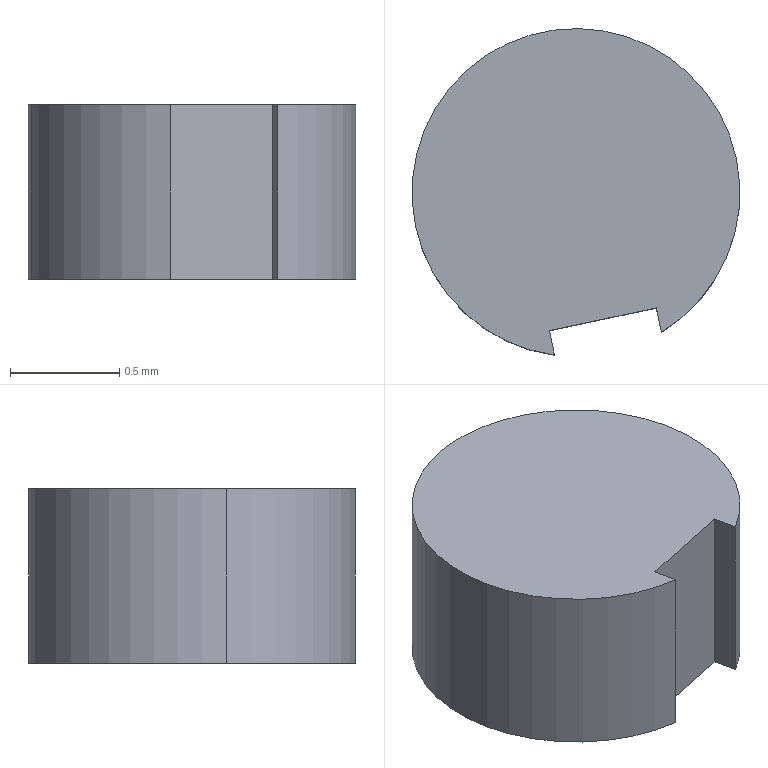Component | SolidWorks | Part32^Assembly1-2 | 1 solid | 8 faces | box 1.5 x 1.49 x 0.8 mm | volume 1 mm3 | plane 5 | cylinder 3 | commonest cylinder face diameters 1.5 x3
STEP:
#1=COLOUR_RGB('',0.7922,0.8196,0.9333);
#2=FILL_AREA_STYLE_COLOUR('',#1);
#3=FILL_AREA_STYLE('',(#2));
#4=SURFACE_STYLE_FILL_AREA(#3);
#5=SURFACE_SIDE_STYLE('',(#4));
#6=SURFACE_STYLE_USAGE(.BOTH.,#5);
#7=PRESENTATION_STYLE_ASSIGNMENT((#6));
#8=CARTESIAN_POINT('',(0.2553,-0.1317,0.1895));
#9=VERTEX_POINT('',#8);
#10=CARTESIAN_POINT('',(0.1975,-0.1439,0.1895));
#11=VERTEX_POINT('',#10);
#12=CARTESIAN_POINT('',(0.2264,-0.1378,0.1895));
#13=DIRECTION('',(0.,-0.,1.));
#14=DIRECTION('',(0.9782,0.2075,0.));
#15=AXIS2_PLACEMENT_3D('',#12,#13,#14);
#16=CIRCLE('',#15,0.02953);
#17=EDGE_CURVE('',#9,#11,#16,.T.);
#18=ORIENTED_EDGE('',*,*,#17,.F.);
#19=CARTESIAN_POINT('',(0.2553,-0.1317,0.158));
#20=VERTEX_POINT('',#19);
#21=CARTESIAN_POINT('',(0.2553,-0.1317,0.1895));
#22=DIRECTION('',(-0.,0.,-1.));
#23=VECTOR('',#22,39.37);
#24=LINE('',#21,#23);
#25=EDGE_CURVE('',#9,#20,#24,.T.);
#26=ORIENTED_EDGE('',*,*,#25,.T.);
#27=CARTESIAN_POINT('',(0.1975,-0.1439,0.158));
#28=VERTEX_POINT('',#27);
#29=CARTESIAN_POINT('',(0.2264,-0.1378,0.158));
#30=DIRECTION('',(0.,-0.,1.));
#31=DIRECTION('',(0.9782,0.2075,0.));
#32=AXIS2_PLACEMENT_3D('',#29,#30,#31);
#33=CIRCLE('',#32,0.02953);
#34=EDGE_CURVE('',#20,#28,#33,.T.);
#35=ORIENTED_EDGE('',*,*,#34,.T.);
#36=CARTESIAN_POINT('',(0.1975,-0.1439,0.1895));
#37=DIRECTION('',(-0.,0.,-1.));
#38=VECTOR('',#37,39.37);
#39=LINE('',#36,#38);
#40=EDGE_CURVE('',#11,#28,#39,.T.);
#41=ORIENTED_EDGE('',*,*,#40,.F.);
#42=EDGE_LOOP('',(#18,#26,#35,#41));
#43=FACE_OUTER_BOUND('',#42,.T.);
#44=CARTESIAN_POINT('',(0.2264,-0.1378,0.1895));
#45=DIRECTION('',(-0.,0.,-1.));
#46=DIRECTION('',(-0.9782,-0.2075,0.));
#47=AXIS2_PLACEMENT_3D('',#44,#45,#46);
#48=CYLINDRICAL_SURFACE('',#47,0.02953);
#49=ADVANCED_FACE('',(#43),#48,.T.);
#50=CARTESIAN_POINT('',(0.2225,-0.1671,0.1895));
#51=VERTEX_POINT('',#50);
#52=CARTESIAN_POINT('',(0.2264,-0.1378,0.1895));
#53=DIRECTION('',(0.,-0.,1.));
#54=DIRECTION('',(0.9782,0.2075,0.));
#55=AXIS2_PLACEMENT_3D('',#52,#53,#54);
#56=CIRCLE('',#55,0.02953);
#57=EDGE_CURVE('',#11,#51,#56,.T.);
#58=ORIENTED_EDGE('',*,*,#57,.F.);
#59=ORIENTED_EDGE('',*,*,#40,.T.);
#60=CARTESIAN_POINT('',(0.2225,-0.1671,0.158));
#61=VERTEX_POINT('',#60);
#62=CARTESIAN_POINT('',(0.2264,-0.1378,0.158));
#63=DIRECTION('',(0.,-0.,1.));
#64=DIRECTION('',(0.9782,0.2075,0.));
#65=AXIS2_PLACEMENT_3D('',#62,#63,#64);
#66=CIRCLE('',#65,0.02953);
#67=EDGE_CURVE('',#28,#61,#66,.T.);
#68=ORIENTED_EDGE('',*,*,#67,.T.);
#69=CARTESIAN_POINT('',(0.2225,-0.1671,0.1895));
#70=DIRECTION('',(-0.,0.,-1.));
#71=VECTOR('',#70,39.37);
#72=LINE('',#69,#71);
#73=EDGE_CURVE('',#51,#61,#72,.T.);
#74=ORIENTED_EDGE('',*,*,#73,.F.);
#75=EDGE_LOOP('',(#58,#59,#68,#74));
#76=FACE_OUTER_BOUND('',#75,.T.);
#77=CARTESIAN_POINT('',(0.2264,-0.1378,0.1895));
#78=DIRECTION('',(-0.,0.,-1.));
#79=DIRECTION('',(-0.9782,-0.2075,0.));
#80=AXIS2_PLACEMENT_3D('',#77,#78,#79);
#81=CYLINDRICAL_SURFACE('',#80,0.02953);
#82=ADVANCED_FACE('',(#76),#81,.T.);
#83=CARTESIAN_POINT('',(0.2418,-0.163,0.158));
#84=VERTEX_POINT('',#83);
#85=CARTESIAN_POINT('',(0.2408,-0.1586,0.158));
#86=VERTEX_POINT('',#85);
#87=CARTESIAN_POINT('',(0.236,-0.1358,0.158));
#88=DIRECTION('',(-0.2075,0.9782,0.));
#89=VECTOR('',#88,39.37);
#90=LINE('',#87,#89);
#91=EDGE_CURVE('',#84,#86,#90,.T.);
#92=ORIENTED_EDGE('',*,*,#91,.F.);
#93=CARTESIAN_POINT('',(0.2418,-0.163,0.1895));
#94=VERTEX_POINT('',#93);
#95=CARTESIAN_POINT('',(0.2418,-0.163,0.1895));
#96=DIRECTION('',(-0.,0.,-1.));
#97=VECTOR('',#96,39.37);
#98=LINE('',#95,#97);
#99=EDGE_CURVE('',#94,#84,#98,.T.);
#100=ORIENTED_EDGE('',*,*,#99,.F.);
#101=CARTESIAN_POINT('',(0.2408,-0.1586,0.1895));
#102=VERTEX_POINT('',#101);
#103=CARTESIAN_POINT('',(0.236,-0.1358,0.1895));
#104=DIRECTION('',(-0.2075,0.9782,0.));
#105=VECTOR('',#104,39.37);
#106=LINE('',#103,#105);
#107=EDGE_CURVE('',#94,#102,#106,.T.);
#108=ORIENTED_EDGE('',*,*,#107,.T.);
#109=CARTESIAN_POINT('',(0.2408,-0.1586,0.1895));
#110=DIRECTION('',(-0.,0.,-1.));
#111=VECTOR('',#110,39.37);
#112=LINE('',#109,#111);
#113=EDGE_CURVE('',#102,#86,#112,.T.);
#114=ORIENTED_EDGE('',*,*,#113,.T.);
#115=EDGE_LOOP('',(#92,#100,#108,#114));
#116=FACE_OUTER_BOUND('',#115,.T.);
#117=CARTESIAN_POINT('',(0.236,-0.1358,0.1895));
#118=DIRECTION('',(-0.9782,-0.2075,0.));
#119=DIRECTION('',(0.,-0.,1.));
#120=AXIS2_PLACEMENT_3D('',#117,#118,#119);
#121=PLANE('',#120);
#122=ADVANCED_FACE('',(#116),#121,.T.);
#123=ORIENTED_EDGE('',*,*,#25,.F.);
#124=CARTESIAN_POINT('',(0.2264,-0.1378,0.1895));
#125=DIRECTION('',(0.,-0.,1.));
#126=DIRECTION('',(0.9782,0.2075,0.));
#127=AXIS2_PLACEMENT_3D('',#124,#125,#126);
#128=CIRCLE('',#127,0.02953);
#129=EDGE_CURVE('',#94,#9,#128,.T.);
#130=ORIENTED_EDGE('',*,*,#129,.F.);
#131=ORIENTED_EDGE('',*,*,#99,.T.);
#132=CARTESIAN_POINT('',(0.2264,-0.1378,0.158));
#133=DIRECTION('',(0.,-0.,1.));
#134=DIRECTION('',(0.9782,0.2075,0.));
#135=AXIS2_PLACEMENT_3D('',#132,#133,#134);
#136=CIRCLE('',#135,0.02953);
#137=EDGE_CURVE('',#84,#20,#136,.T.);
#138=ORIENTED_EDGE('',*,*,#137,.T.);
#139=EDGE_LOOP('',(#123,#130,#131,#138));
#140=FACE_OUTER_BOUND('',#139,.T.);
#141=CARTESIAN_POINT('',(0.2264,-0.1378,0.1895));
#142=DIRECTION('',(-0.,0.,-1.));
#143=DIRECTION('',(-0.9782,-0.2075,0.));
#144=AXIS2_PLACEMENT_3D('',#141,#142,#143);
#145=CYLINDRICAL_SURFACE('',#144,0.02953);
#146=ADVANCED_FACE('',(#140),#145,.T.);
#147=CARTESIAN_POINT('',(0.2216,-0.1627,0.158));
#148=VERTEX_POINT('',#147);
#149=CARTESIAN_POINT('',(0.2167,-0.1398,0.158));
#150=DIRECTION('',(-0.2075,0.9782,0.));
#151=VECTOR('',#150,39.37);
#152=LINE('',#149,#151);
#153=EDGE_CURVE('',#61,#148,#152,.T.);
#154=ORIENTED_EDGE('',*,*,#153,.T.);
#155=CARTESIAN_POINT('',(0.2216,-0.1627,0.1895));
#156=VERTEX_POINT('',#155);
#157=CARTESIAN_POINT('',(0.2216,-0.1627,0.1895));
#158=DIRECTION('',(-0.,0.,-1.));
#159=VECTOR('',#158,39.37);
#160=LINE('',#157,#159);
#161=EDGE_CURVE('',#156,#148,#160,.T.);
#162=ORIENTED_EDGE('',*,*,#161,.F.);
#163=CARTESIAN_POINT('',(0.2167,-0.1398,0.1895));
#164=DIRECTION('',(-0.2075,0.9782,0.));
#165=VECTOR('',#164,39.37);
#166=LINE('',#163,#165);
#167=EDGE_CURVE('',#51,#156,#166,.T.);
#168=ORIENTED_EDGE('',*,*,#167,.F.);
#169=ORIENTED_EDGE('',*,*,#73,.T.);
#170=EDGE_LOOP('',(#154,#162,#168,#169));
#171=FACE_OUTER_BOUND('',#170,.T.);
#172=CARTESIAN_POINT('',(0.2167,-0.1398,0.1895));
#173=DIRECTION('',(-0.9782,-0.2075,0.));
#174=DIRECTION('',(0.,-0.,1.));
#175=AXIS2_PLACEMENT_3D('',#172,#173,#174);
#176=PLANE('',#175);
#177=ADVANCED_FACE('',(#171),#176,.F.);
#178=CARTESIAN_POINT('',(0.2312,-0.1606,0.158));
#179=DIRECTION('',(-0.9782,-0.2075,0.));
#180=VECTOR('',#179,39.37);
#181=LINE('',#178,#180);
#182=EDGE_CURVE('',#86,#148,#181,.T.);
#183=ORIENTED_EDGE('',*,*,#182,.F.);
#184=ORIENTED_EDGE('',*,*,#113,.F.);
#185=CARTESIAN_POINT('',(0.2312,-0.1606,0.1895));
#186=DIRECTION('',(-0.9782,-0.2075,0.));
#187=VECTOR('',#186,39.37);
#188=LINE('',#185,#187);
#189=EDGE_CURVE('',#102,#156,#188,.T.);
#190=ORIENTED_EDGE('',*,*,#189,.T.);
#191=ORIENTED_EDGE('',*,*,#161,.T.);
#192=EDGE_LOOP('',(#183,#184,#190,#191));
#193=FACE_OUTER_BOUND('',#192,.T.);
#194=CARTESIAN_POINT('',(0.2312,-0.1606,0.1895));
#195=DIRECTION('',(0.2075,-0.9782,-0.));
#196=DIRECTION('',(-0.,0.,-1.));
#197=AXIS2_PLACEMENT_3D('',#194,#195,#196);
#198=PLANE('',#197);
#199=ADVANCED_FACE('',(#193),#198,.T.);
#200=ORIENTED_EDGE('',*,*,#107,.F.);
#201=ORIENTED_EDGE('',*,*,#129,.T.);
#202=ORIENTED_EDGE('',*,*,#17,.T.);
#203=ORIENTED_EDGE('',*,*,#57,.T.);
#204=ORIENTED_EDGE('',*,*,#167,.T.);
#205=ORIENTED_EDGE('',*,*,#189,.F.);
#206=EDGE_LOOP('',(#200,#201,#202,#203,#204,#205));
#207=FACE_OUTER_BOUND('',#206,.T.);
#208=CARTESIAN_POINT('',(0.2264,-0.1378,0.1895));
#209=DIRECTION('',(0.,-0.,1.));
#210=DIRECTION('',(0.9782,0.2075,-0.));
#211=AXIS2_PLACEMENT_3D('',#208,#209,#210);
#212=PLANE('',#211);
#213=ADVANCED_FACE('',(#207),#212,.T.);
#214=ORIENTED_EDGE('',*,*,#91,.T.);
#215=ORIENTED_EDGE('',*,*,#182,.T.);
#216=ORIENTED_EDGE('',*,*,#153,.F.);
#217=ORIENTED_EDGE('',*,*,#67,.F.);
#218=ORIENTED_EDGE('',*,*,#34,.F.);
#219=ORIENTED_EDGE('',*,*,#137,.F.);
#220=EDGE_LOOP('',(#214,#215,#216,#217,#218,#219));
#221=FACE_OUTER_BOUND('',#220,.T.);
#222=CARTESIAN_POINT('',(0.2264,-0.1378,0.158));
#223=DIRECTION('',(0.,-0.,1.));
#224=DIRECTION('',(0.9782,0.2075,-0.));
#225=AXIS2_PLACEMENT_3D('',#222,#223,#224);
#226=PLANE('',#225);
#227=ADVANCED_FACE('',(#221),#226,.F.);
#228=CLOSED_SHELL('',(#49,#82,#122,#146,#177,#199,#213,#227));
#229=MANIFOLD_SOLID_BREP('',#228);
#230=STYLED_ITEM('',(#7),#229);
#231=PRESENTATION_LAYER_ASSIGNMENT('','',(#230));
#232=CARTESIAN_POINT('',(0.,0.,0.));
#233=DIRECTION('',(0.,0.,1.));
#234=DIRECTION('',(1.,0.,0.));
#235=AXIS2_PLACEMENT_3D('',#232,#233,#234);
#236=(LENGTH_UNIT()NAMED_UNIT(*)SI_UNIT($,.METRE.));
#237=LENGTH_MEASURE_WITH_UNIT(LENGTH_MEASURE(0.0254),#236);
#238=DIMENSIONAL_EXPONENTS(1.,0.,0.,0.,0.,0.,0.);
#239=(CONVERSION_BASED_UNIT('',#237)LENGTH_UNIT()NAMED_UNIT(#238));
#240=UNCERTAINTY_MEASURE_WITH_UNIT(LENGTH_MEASURE(0.00001),#239,'','');
#241=(NAMED_UNIT(*)PLANE_ANGLE_UNIT()SI_UNIT($,.RADIAN.));
#242=(NAMED_UNIT(*)SI_UNIT($,.STERADIAN.)SOLID_ANGLE_UNIT());
#243=(GEOMETRIC_REPRESENTATION_CONTEXT(3)GLOBAL_UNCERTAINTY_ASSIGNED_CONTEXT((#240))GLOBAL_UNIT_ASSIGNED_CONTEXT((#239,#241,#242))REPRESENTATION_CONTEXT('',''));
#244=ADVANCED_BREP_SHAPE_REPRESENTATION('',(#229,#235),#243);
#245=(LENGTH_UNIT()NAMED_UNIT(*)SI_UNIT($,.METRE.));
#246=LENGTH_MEASURE_WITH_UNIT(LENGTH_MEASURE(0.0254),#245);
#247=DIMENSIONAL_EXPONENTS(1.,0.,0.,0.,0.,0.,0.);
#248=(CONVERSION_BASED_UNIT('',#246)LENGTH_UNIT()NAMED_UNIT(#247));
#249=UNCERTAINTY_MEASURE_WITH_UNIT(LENGTH_MEASURE(0.00001),#248,'','');
#250=(NAMED_UNIT(*)PLANE_ANGLE_UNIT()SI_UNIT($,.RADIAN.));
#251=(NAMED_UNIT(*)SI_UNIT($,.STERADIAN.)SOLID_ANGLE_UNIT());
#252=(GEOMETRIC_REPRESENTATION_CONTEXT(3)GLOBAL_UNCERTAINTY_ASSIGNED_CONTEXT((#249))GLOBAL_UNIT_ASSIGNED_CONTEXT((#248,#250,#251))REPRESENTATION_CONTEXT('',''));
#253=MECHANICAL_DESIGN_GEOMETRIC_PRESENTATION_REPRESENTATION('',(#230),#252);